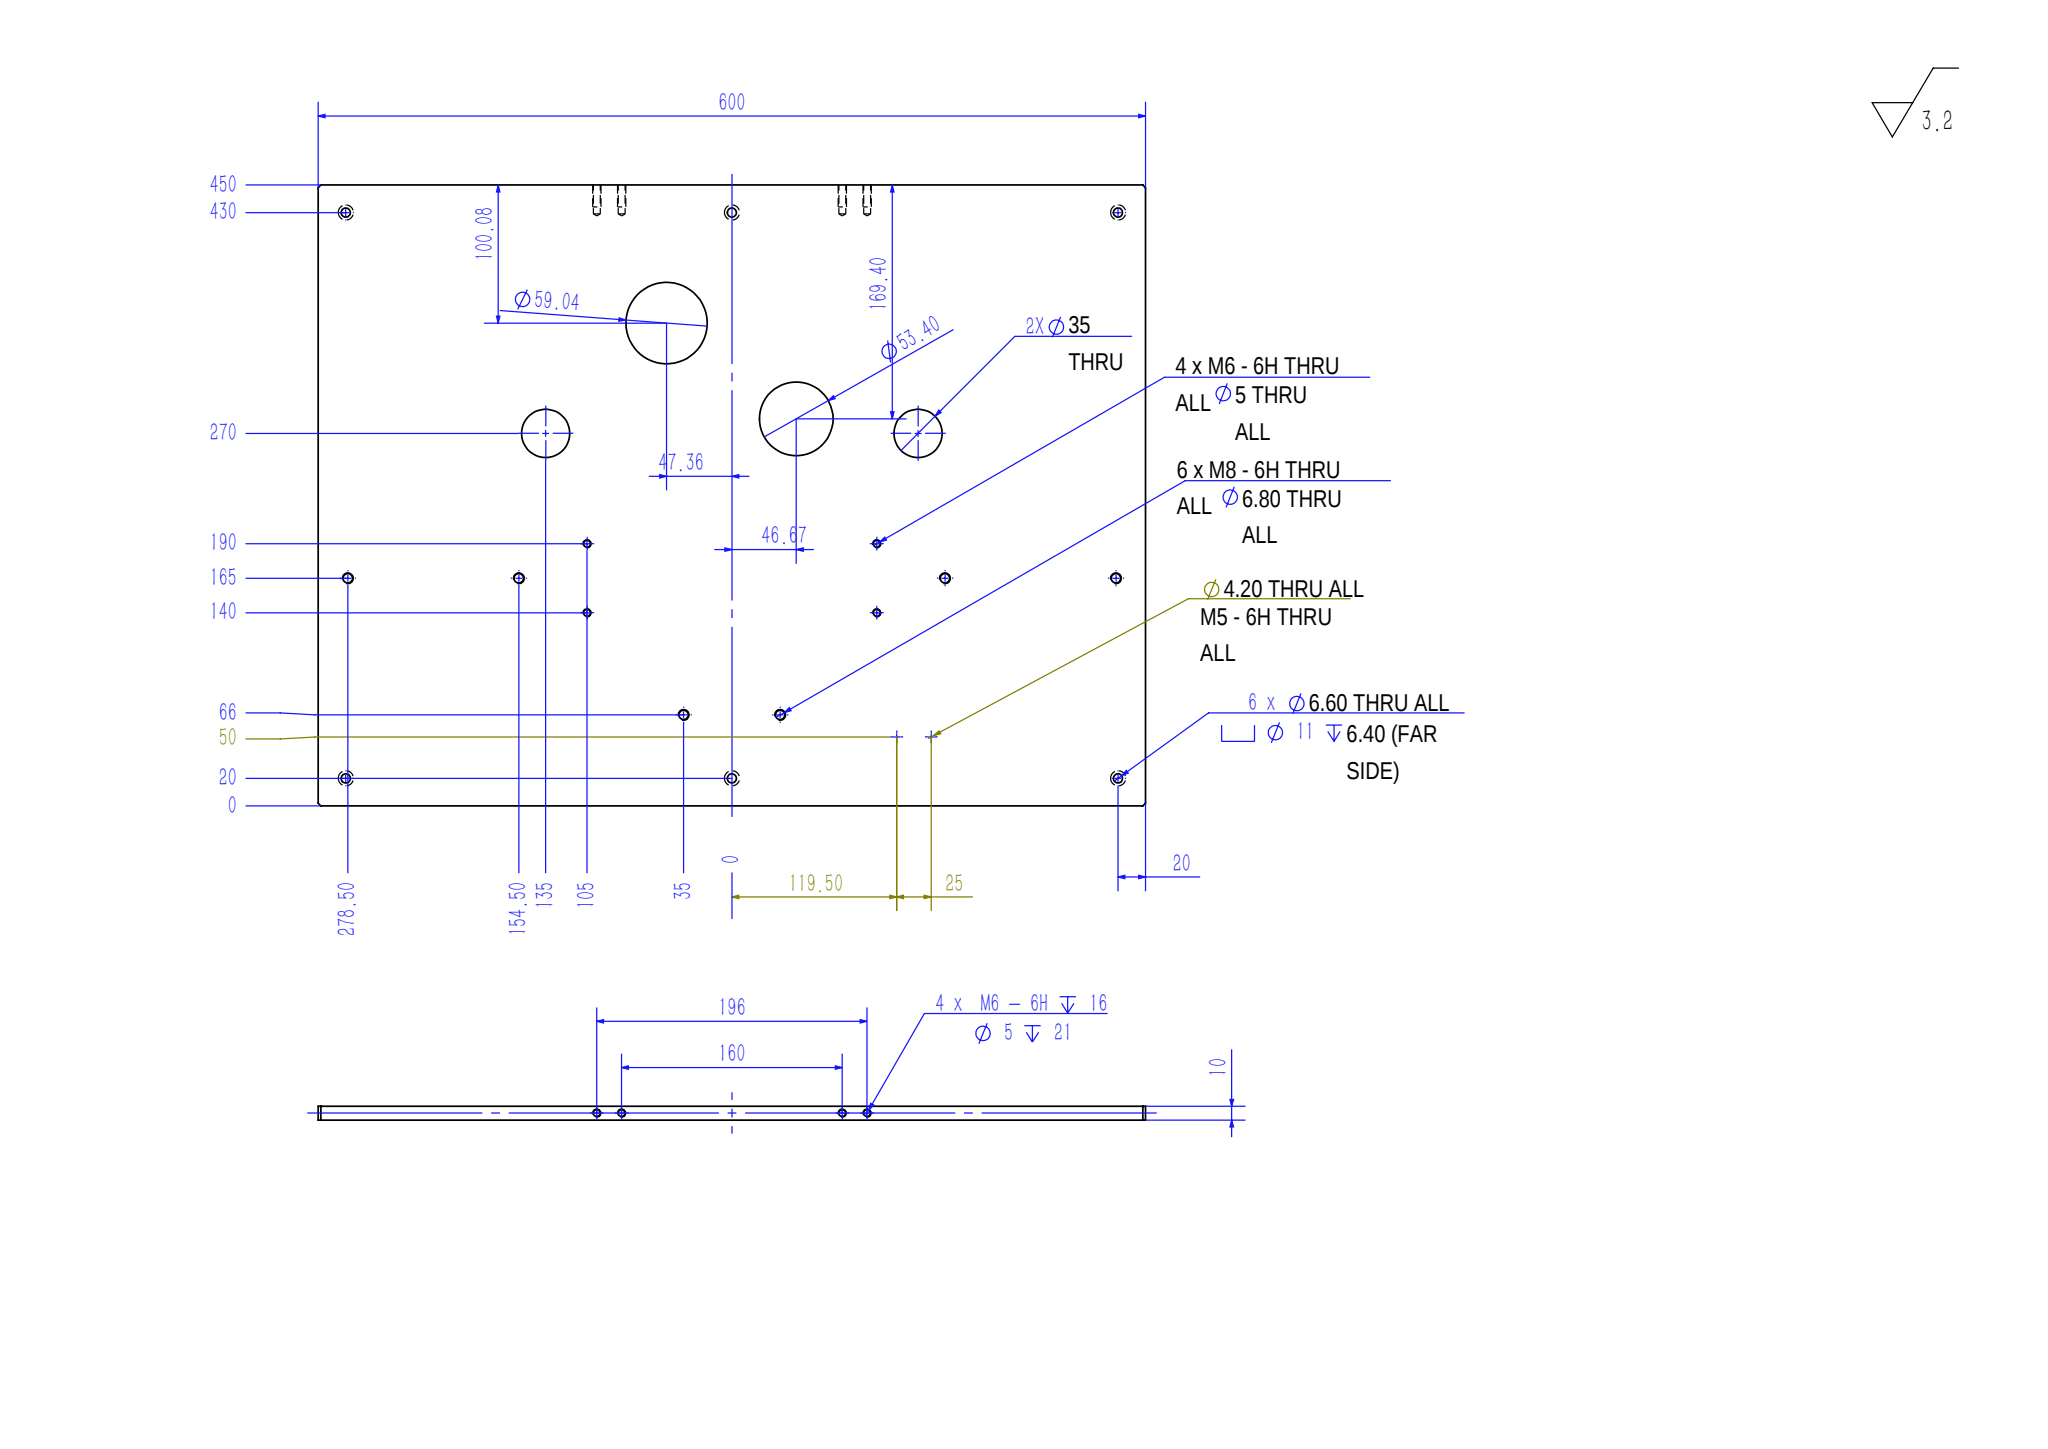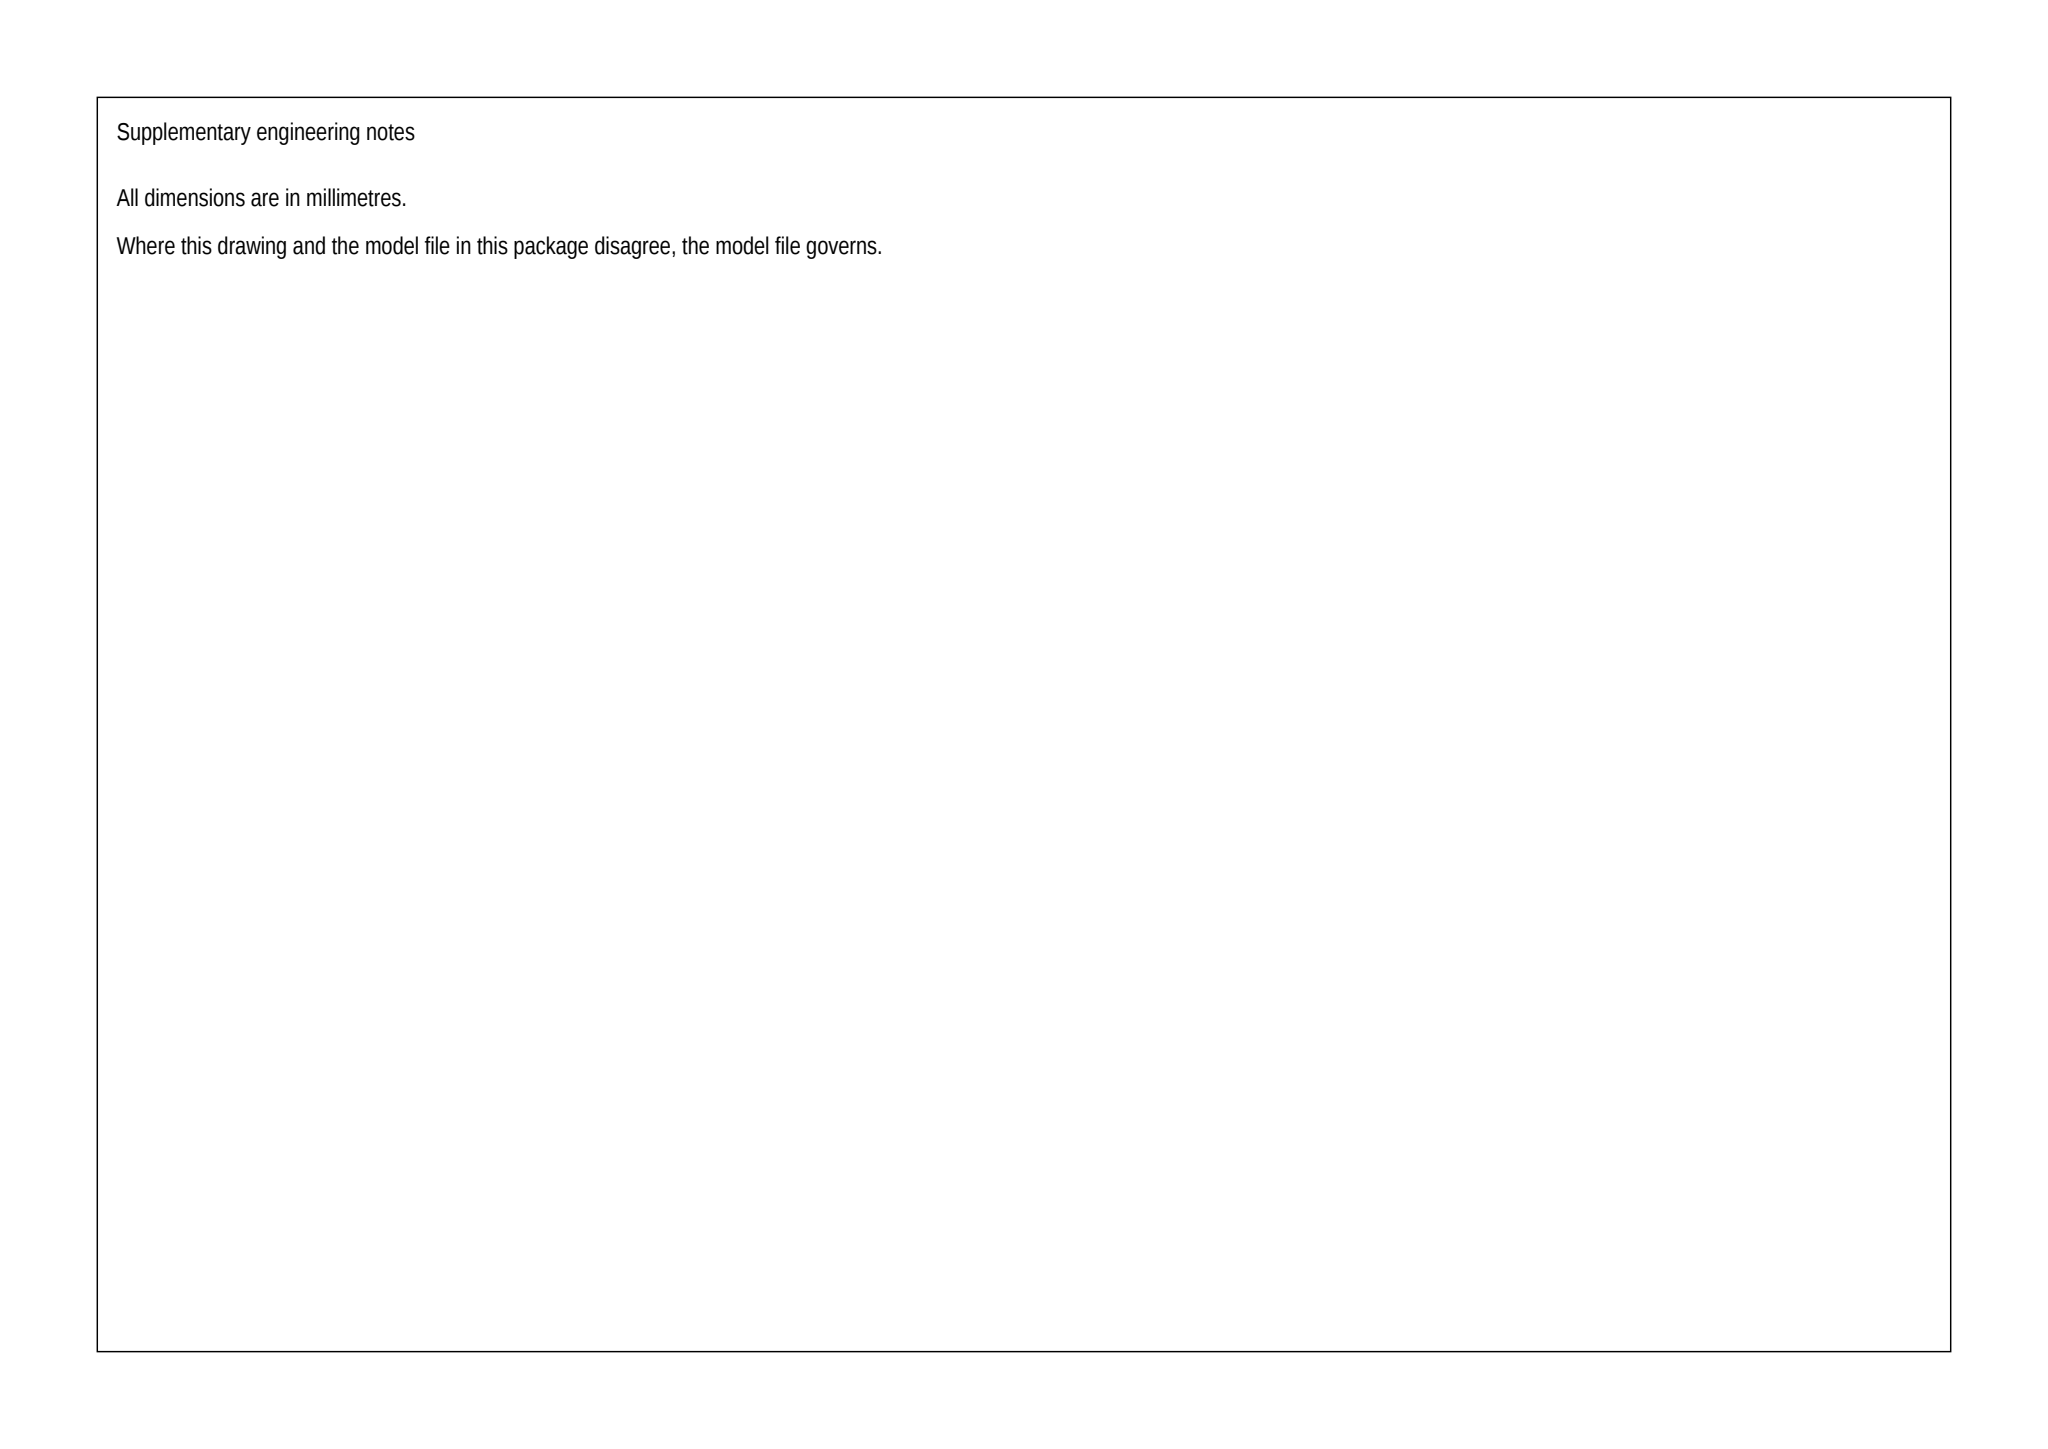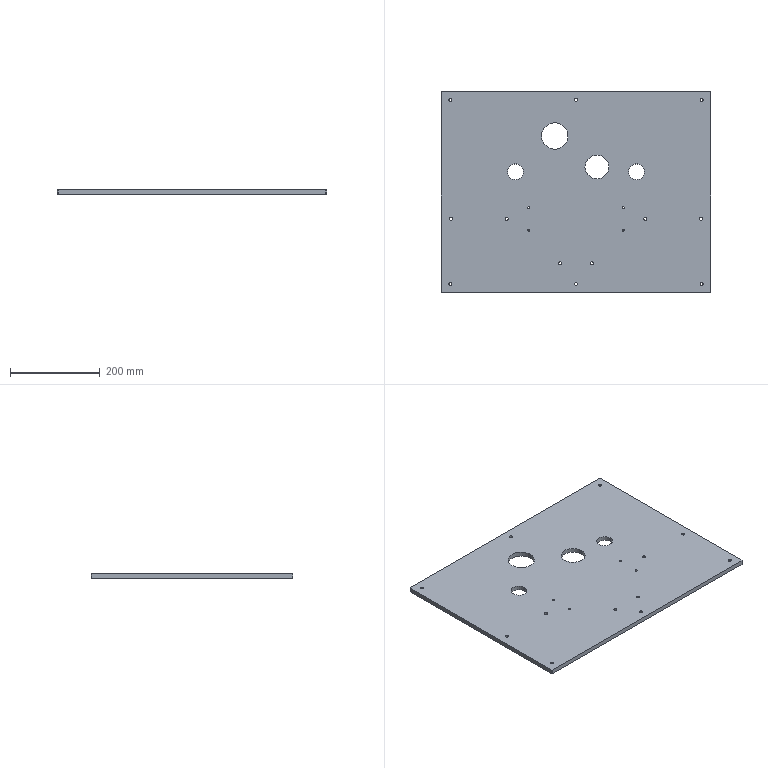Part | SolidWorks | mm | 1 solid | 84 faces | box 600 x 450 x 10 mm | volume 2621863 mm3 | cylinder 60 | plane 16 | cone 8 | commonest cylinder face diameters 5 x16 6.8 x12 11 x12 6.6 x12 35 x4 59.044 x2 53.396 x2
build123d program:
from build123d import *

# Parameters (mm, degrees)
SKETCH1_W                                       = 600
SKETCH1_H                                       = 450
BOSS_EXTRUDE1_DEPTH                             = 10
M6_HEX_SOCKET_HEAD_CAP_SCREW_CBORE1_D           = 6.6
M6_HEX_SOCKET_HEAD_CAP_SCREW_CBORE1_CBORE_D     = 11
M6_HEX_SOCKET_HEAD_CAP_SCREW_CBORE1_CBORE_DEPTH = 6.4
M8_TAPPED_HOLE1_D                               = 6.8
M6_TAPPED_HOLE1_D                               = 5
M6_TAPPED_HOLE2_D                               = 5
M6_TAPPED_HOLE2_DEPTH                           = 21
M6_TAPPED_HOLE2_TIP                             = 1.502
SKETCH21_R                                      = 17.5
CUT_EXTRUDE1_DEPTH                              = 12
CHAMFER1_SIZE                                   = 2
SKETCH22_R                                      = 29.522
SKETCH22_R_2                                    = 26.698
CUT_EXTRUDE2_DEPTH                              = 80


with BuildPart() as part:
    # Sketch1 → Boss-Extrude1 (new body)
    with BuildSketch(Plane.XY):
        Rectangle(SKETCH1_W, SKETCH1_H)
    extrude(amount=BOSS_EXTRUDE1_DEPTH)

    # M6 Hex Socket Head Cap Screw CBORE1 (through all)
    with Locations(Plane(origin=(0, 0, 0), x_dir=(-1, 0, 0), z_dir=(0, 0, -1))):
        with Locations((280, -205), (-280, -205), (280, 205), (-280, 205), (0, -205), (0, 205)):
            CounterBoreHole(M6_HEX_SOCKET_HEAD_CAP_SCREW_CBORE1_D / 2, M6_HEX_SOCKET_HEAD_CAP_SCREW_CBORE1_CBORE_D / 2, M6_HEX_SOCKET_HEAD_CAP_SCREW_CBORE1_CBORE_DEPTH)

    # M8 Tapped Hole1 (through all)
    with Locations(Plane(origin=(35, -159, 0), x_dir=(-1, 0, 0), z_dir=(0, 0, -1))):
        with Locations((0, 0), (70, 0), (-243.5, 99), (-119.5, 99), (189.5, 99), (313.5, 99)):
            Hole(M8_TAPPED_HOLE1_D / 2)

    # M6 Tapped Hole1 (through all)
    with Locations(Plane(origin=(0, 0, 0), x_dir=(-1, 0, 0), z_dir=(0, 0, -1))):
        with Locations((-105, -35), (105, -35), (-105, -85), (105, -85)):
            Hole(M6_TAPPED_HOLE1_D / 2)

    # M6 Tapped Hole2
    with Locations(Plane(origin=(0, 225, 0), x_dir=(1, 0, 0), z_dir=(0, 1, 0))):
        with Locations((-98, -5), (-80, -5), (80, -5), (98, -5)):
            Hole(M6_TAPPED_HOLE2_D / 2, depth=M6_TAPPED_HOLE2_DEPTH)
            with Locations((0, 0, -(M6_TAPPED_HOLE2_DEPTH + M6_TAPPED_HOLE2_TIP / 2))):  # 118° drill point
                Cone(0, M6_TAPPED_HOLE2_D / 2, M6_TAPPED_HOLE2_TIP, mode=Mode.SUBTRACT)

    # Sketch21 → Cut-Extrude1 (cut)
    with BuildSketch(Plane(origin=(0, 0, 0), x_dir=(-1, 0, 0), z_dir=(0, 0, -1))):
        with Locations((135, 45)):
            Circle(SKETCH21_R)
        with Locations((-135, 45)):
            Circle(SKETCH21_R)
    extrude(amount=-CUT_EXTRUDE1_DEPTH, mode=Mode.SUBTRACT)

    # Chamfer1
    chamfer1_edges = [part.edges().sort_by_distance(p)[0] for p in [
        (300, -225, 5),
        (-300, -225, 5),
        (-300, 225, 5),
        (300, 225, 5),
    ]]
    chamfer(chamfer1_edges, length=CHAMFER1_SIZE)

    # Sketch22 → Cut-Extrude2 (cut)
    with BuildSketch(Plane(origin=(0, 0, 0), x_dir=(-1, 0, 0), z_dir=(0, 0, -1))):
        with Locations((47.36, 124.92)):
            Circle(SKETCH22_R)
        with Locations((-46.673, 55.596)):
            Circle(SKETCH22_R_2)
    extrude(amount=-CUT_EXTRUDE2_DEPTH, mode=Mode.SUBTRACT)


solid = part.part